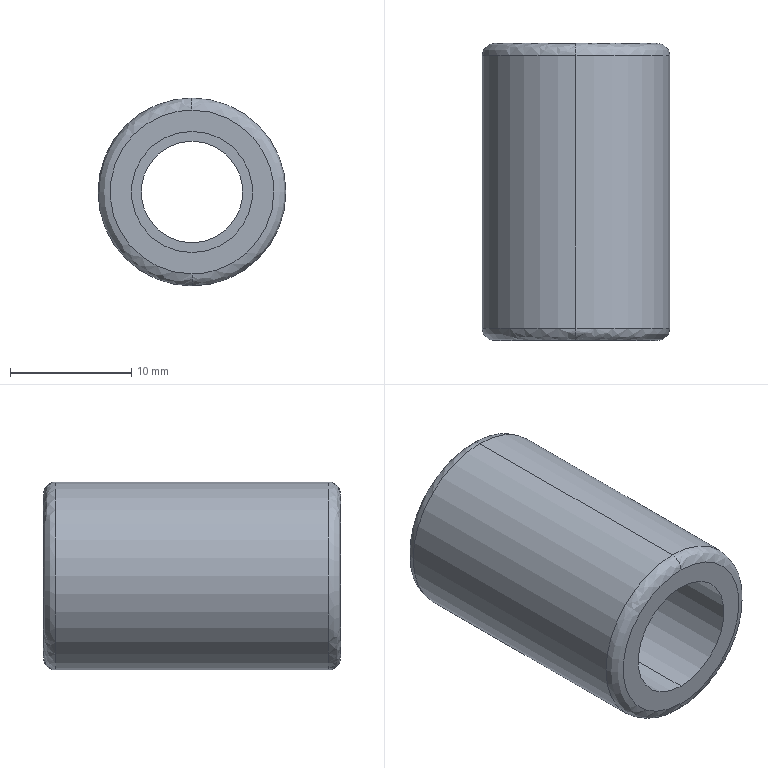Component | SolidWorks | SC-80x75(000)-1_11-1 | 1 solid | 27 faces | box 15.5 x 24.5 x 15.5 mm | volume 2654 mm3 | plane 15 | cylinder 6 | spline 4 | cone 2 | commonest cylinder face diameters 10 x2 15.5 x2 8.376 x2
STEP:
#1=COLOUR_RGB('',0.7922,0.8196,0.9333);
#2=FILL_AREA_STYLE_COLOUR('',#1);
#3=FILL_AREA_STYLE('',(#2));
#4=SURFACE_STYLE_FILL_AREA(#3);
#5=SURFACE_SIDE_STYLE('',(#4));
#6=SURFACE_STYLE_USAGE(.BOTH.,#5);
#7=PRESENTATION_STYLE_ASSIGNMENT((#6));
#8=CARTESIAN_POINT('',(-0.5951,7.131,9.518));
#9=VERTEX_POINT('',#8);
#10=CARTESIAN_POINT('',(-0.5951,7.131,8.986));
#11=VERTEX_POINT('',#10);
#12=CARTESIAN_POINT('',(-0.5951,7.131,9.518));
#13=CARTESIAN_POINT('',(-1.127,7.131,9.518));
#14=CARTESIAN_POINT('',(-1.127,7.131,8.986));
#15=CARTESIAN_POINT('',(-0.5951,7.131,8.986));
#16=(BOUNDED_CURVE()B_SPLINE_CURVE(3,(#12,#13,#14,#15),.UNSPECIFIED.,.F.,.F.)B_SPLINE_CURVE_WITH_KNOTS((4,4),(0.,1.),.UNSPECIFIED.)CURVE()GEOMETRIC_REPRESENTATION_ITEM()RATIONAL_B_SPLINE_CURVE((1.,0.3333,0.3333,1.))REPRESENTATION_ITEM(''));
#17=EDGE_CURVE('',#9,#11,#16,.T.);
#18=ORIENTED_EDGE('',*,*,#17,.T.);
#19=CARTESIAN_POINT('',(-0.5951,7.092,8.947));
#20=VERTEX_POINT('',#19);
#21=CARTESIAN_POINT('',(-0.5951,7.092,8.986));
#22=DIRECTION('',(-1.,-0.,-0.));
#23=DIRECTION('',(0.,0.,-1.));
#24=AXIS2_PLACEMENT_3D('',#21,#22,#23);
#25=CIRCLE('',#24,0.03937);
#26=EDGE_CURVE('',#11,#20,#25,.T.);
#27=ORIENTED_EDGE('',*,*,#26,.T.);
#28=CARTESIAN_POINT('',(-0.5951,7.092,9.557));
#29=VERTEX_POINT('',#28);
#30=CARTESIAN_POINT('',(-0.5951,7.092,9.252));
#31=DIRECTION('',(0.,-1.,0.));
#32=DIRECTION('',(-0.,0.,1.));
#33=AXIS2_PLACEMENT_3D('',#30,#31,#32);
#34=CIRCLE('',#33,0.3051);
#35=EDGE_CURVE('',#29,#20,#34,.T.);
#36=ORIENTED_EDGE('',*,*,#35,.F.);
#37=CARTESIAN_POINT('',(-0.5951,7.092,9.518));
#38=DIRECTION('',(1.,0.,0.));
#39=DIRECTION('',(0.,0.,1.));
#40=AXIS2_PLACEMENT_3D('',#37,#38,#39);
#41=CIRCLE('',#40,0.03937);
#42=EDGE_CURVE('',#9,#29,#41,.T.);
#43=ORIENTED_EDGE('',*,*,#42,.F.);
#44=EDGE_LOOP('',(#18,#27,#36,#43));
#45=FACE_OUTER_BOUND('',#44,.T.);
#46=CARTESIAN_POINT('',(-0.5951,7.131,8.986));
#47=CARTESIAN_POINT('',(-1.127,7.131,8.986));
#48=CARTESIAN_POINT('',(-1.127,7.131,9.518));
#49=CARTESIAN_POINT('',(-0.5951,7.131,9.518));
#50=CARTESIAN_POINT('',(-0.5951,7.131,8.963));
#51=CARTESIAN_POINT('',(-1.173,7.131,8.963));
#52=CARTESIAN_POINT('',(-1.173,7.131,9.541));
#53=CARTESIAN_POINT('',(-0.5951,7.131,9.541));
#54=CARTESIAN_POINT('',(-0.5951,7.115,8.947));
#55=CARTESIAN_POINT('',(-1.205,7.115,8.947));
#56=CARTESIAN_POINT('',(-1.205,7.115,9.557));
#57=CARTESIAN_POINT('',(-0.5951,7.115,9.557));
#58=CARTESIAN_POINT('',(-0.5951,7.092,8.947));
#59=CARTESIAN_POINT('',(-1.205,7.092,8.947));
#60=CARTESIAN_POINT('',(-1.205,7.092,9.557));
#61=CARTESIAN_POINT('',(-0.5951,7.092,9.557));
#62=(BOUNDED_SURFACE()B_SPLINE_SURFACE(3,3,((#46,#47,#48,#49),(#50,#51,#52,#53),(#54,#55,#56,#57),(#58,#59,#60,#61)),.UNSPECIFIED.,.F.,.F.,.T.)B_SPLINE_SURFACE_WITH_KNOTS((4,4),(4,4),(0.,1.),(0.,1.),.UNSPECIFIED.)GEOMETRIC_REPRESENTATION_ITEM()RATIONAL_B_SPLINE_SURFACE(((1.,0.3333,0.3333,1.),(0.8047,0.2682,0.2682,0.8047),(0.8047,0.2682,0.2682,0.8047),(1.,0.3333,0.3333,1.)))REPRESENTATION_ITEM('')SURFACE());
#63=ADVANCED_FACE('',(#45),#62,.T.);
#64=CARTESIAN_POINT('',(-0.5951,6.206,8.947));
#65=VERTEX_POINT('',#64);
#66=CARTESIAN_POINT('',(-0.5951,6.206,9.557));
#67=VERTEX_POINT('',#66);
#68=CARTESIAN_POINT('',(-0.5951,6.206,9.252));
#69=DIRECTION('',(-0.,1.,-0.));
#70=DIRECTION('',(-0.,0.,1.));
#71=AXIS2_PLACEMENT_3D('',#68,#69,#70);
#72=CIRCLE('',#71,0.3051);
#73=EDGE_CURVE('',#65,#67,#72,.T.);
#74=ORIENTED_EDGE('',*,*,#73,.F.);
#75=CARTESIAN_POINT('',(-0.5951,6.167,8.986));
#76=VERTEX_POINT('',#75);
#77=CARTESIAN_POINT('',(-0.5951,6.206,8.986));
#78=DIRECTION('',(-1.,-0.,-0.));
#79=DIRECTION('',(0.,0.,-1.));
#80=AXIS2_PLACEMENT_3D('',#77,#78,#79);
#81=CIRCLE('',#80,0.03937);
#82=EDGE_CURVE('',#65,#76,#81,.T.);
#83=ORIENTED_EDGE('',*,*,#82,.T.);
#84=CARTESIAN_POINT('',(-0.5951,6.167,9.518));
#85=VERTEX_POINT('',#84);
#86=CARTESIAN_POINT('',(-0.5951,6.167,8.986));
#87=CARTESIAN_POINT('',(-1.127,6.167,8.986));
#88=CARTESIAN_POINT('',(-1.127,6.167,9.518));
#89=CARTESIAN_POINT('',(-0.5951,6.167,9.518));
#90=(BOUNDED_CURVE()B_SPLINE_CURVE(3,(#86,#87,#88,#89),.UNSPECIFIED.,.F.,.F.)B_SPLINE_CURVE_WITH_KNOTS((4,4),(0.,1.),.UNSPECIFIED.)CURVE()GEOMETRIC_REPRESENTATION_ITEM()RATIONAL_B_SPLINE_CURVE((1.,0.3333,0.3333,1.))REPRESENTATION_ITEM(''));
#91=EDGE_CURVE('',#76,#85,#90,.T.);
#92=ORIENTED_EDGE('',*,*,#91,.T.);
#93=CARTESIAN_POINT('',(-0.5951,6.206,9.518));
#94=DIRECTION('',(1.,0.,0.));
#95=DIRECTION('',(0.,0.,1.));
#96=AXIS2_PLACEMENT_3D('',#93,#94,#95);
#97=CIRCLE('',#96,0.03937);
#98=EDGE_CURVE('',#67,#85,#97,.T.);
#99=ORIENTED_EDGE('',*,*,#98,.F.);
#100=EDGE_LOOP('',(#74,#83,#92,#99));
#101=FACE_OUTER_BOUND('',#100,.T.);
#102=CARTESIAN_POINT('',(-0.5951,6.206,8.947));
#103=CARTESIAN_POINT('',(-1.205,6.206,8.947));
#104=CARTESIAN_POINT('',(-1.205,6.206,9.557));
#105=CARTESIAN_POINT('',(-0.5951,6.206,9.557));
#106=CARTESIAN_POINT('',(-0.5951,6.183,8.947));
#107=CARTESIAN_POINT('',(-1.205,6.183,8.947));
#108=CARTESIAN_POINT('',(-1.205,6.183,9.557));
#109=CARTESIAN_POINT('',(-0.5951,6.183,9.557));
#110=CARTESIAN_POINT('',(-0.5951,6.167,8.963));
#111=CARTESIAN_POINT('',(-1.173,6.167,8.963));
#112=CARTESIAN_POINT('',(-1.173,6.167,9.541));
#113=CARTESIAN_POINT('',(-0.5951,6.167,9.541));
#114=CARTESIAN_POINT('',(-0.5951,6.167,8.986));
#115=CARTESIAN_POINT('',(-1.127,6.167,8.986));
#116=CARTESIAN_POINT('',(-1.127,6.167,9.518));
#117=CARTESIAN_POINT('',(-0.5951,6.167,9.518));
#118=(BOUNDED_SURFACE()B_SPLINE_SURFACE(3,3,((#102,#103,#104,#105),(#106,#107,#108,#109),(#110,#111,#112,#113),(#114,#115,#116,#117)),.UNSPECIFIED.,.F.,.F.,.T.)B_SPLINE_SURFACE_WITH_KNOTS((4,4),(4,4),(0.,1.),(0.,1.),.UNSPECIFIED.)GEOMETRIC_REPRESENTATION_ITEM()RATIONAL_B_SPLINE_SURFACE(((1.,0.3333,0.3333,1.),(0.8047,0.2682,0.2682,0.8047),(0.8047,0.2682,0.2682,0.8047),(1.,0.3333,0.3333,1.)))REPRESENTATION_ITEM('')SURFACE());
#119=ADVANCED_FACE('',(#101),#118,.T.);
#120=CARTESIAN_POINT('',(-0.5951,6.919,9.449));
#121=VERTEX_POINT('',#120);
#122=CARTESIAN_POINT('',(-0.5951,6.919,9.055));
#123=VERTEX_POINT('',#122);
#124=CARTESIAN_POINT('',(-0.5951,6.919,9.252));
#125=DIRECTION('',(-0.,1.,-0.));
#126=DIRECTION('',(0.,0.,-1.));
#127=AXIS2_PLACEMENT_3D('',#124,#125,#126);
#128=CIRCLE('',#127,0.1969);
#129=EDGE_CURVE('',#121,#123,#128,.T.);
#130=ORIENTED_EDGE('',*,*,#129,.T.);
#131=CARTESIAN_POINT('',(-0.5951,6.167,9.055));
#132=VERTEX_POINT('',#131);
#133=CARTESIAN_POINT('',(-0.5951,6.919,9.055));
#134=DIRECTION('',(0.,-1.,0.));
#135=VECTOR('',#134,39.37);
#136=LINE('',#133,#135);
#137=EDGE_CURVE('',#123,#132,#136,.T.);
#138=ORIENTED_EDGE('',*,*,#137,.T.);
#139=CARTESIAN_POINT('',(-0.5951,6.167,9.449));
#140=VERTEX_POINT('',#139);
#141=CARTESIAN_POINT('',(-0.5951,6.167,9.252));
#142=DIRECTION('',(-0.,1.,-0.));
#143=DIRECTION('',(1.,0.,0.));
#144=AXIS2_PLACEMENT_3D('',#141,#142,#143);
#145=CIRCLE('',#144,0.1969);
#146=EDGE_CURVE('',#140,#132,#145,.T.);
#147=ORIENTED_EDGE('',*,*,#146,.F.);
#148=CARTESIAN_POINT('',(-0.5951,6.919,9.449));
#149=DIRECTION('',(0.,-1.,0.));
#150=VECTOR('',#149,39.37);
#151=LINE('',#148,#150);
#152=EDGE_CURVE('',#121,#140,#151,.T.);
#153=ORIENTED_EDGE('',*,*,#152,.F.);
#154=EDGE_LOOP('',(#130,#138,#147,#153));
#155=FACE_OUTER_BOUND('',#154,.T.);
#156=CARTESIAN_POINT('',(-0.5951,6.919,9.252));
#157=DIRECTION('',(0.,-1.,0.));
#158=DIRECTION('',(-0.,0.,1.));
#159=AXIS2_PLACEMENT_3D('',#156,#157,#158);
#160=CYLINDRICAL_SURFACE('',#159,0.1969);
#161=ADVANCED_FACE('',(#155),#160,.F.);
#162=ORIENTED_EDGE('',*,*,#35,.T.);
#163=CARTESIAN_POINT('',(-0.5951,6.649,8.947));
#164=DIRECTION('',(0.,-1.,0.));
#165=VECTOR('',#164,39.37);
#166=LINE('',#163,#165);
#167=EDGE_CURVE('',#20,#65,#166,.T.);
#168=ORIENTED_EDGE('',*,*,#167,.T.);
#169=ORIENTED_EDGE('',*,*,#73,.T.);
#170=CARTESIAN_POINT('',(-0.5951,6.649,9.557));
#171=DIRECTION('',(0.,-1.,0.));
#172=VECTOR('',#171,39.37);
#173=LINE('',#170,#172);
#174=EDGE_CURVE('',#29,#67,#173,.T.);
#175=ORIENTED_EDGE('',*,*,#174,.F.);
#176=EDGE_LOOP('',(#162,#168,#169,#175));
#177=FACE_OUTER_BOUND('',#176,.T.);
#178=CARTESIAN_POINT('',(-0.5951,6.649,9.252));
#179=DIRECTION('',(0.,-1.,0.));
#180=DIRECTION('',(-0.,0.,1.));
#181=AXIS2_PLACEMENT_3D('',#178,#179,#180);
#182=CYLINDRICAL_SURFACE('',#181,0.3051);
#183=ADVANCED_FACE('',(#177),#182,.T.);
#184=CARTESIAN_POINT('',(-0.5951,6.922,9.087));
#185=VERTEX_POINT('',#184);
#186=CARTESIAN_POINT('',(-0.5951,6.922,9.417));
#187=VERTEX_POINT('',#186);
#188=CARTESIAN_POINT('',(-0.5951,6.922,9.252));
#189=DIRECTION('',(0.,-1.,0.));
#190=DIRECTION('',(-0.,0.,1.));
#191=AXIS2_PLACEMENT_3D('',#188,#189,#190);
#192=CIRCLE('',#191,0.1649);
#193=EDGE_CURVE('',#185,#187,#192,.T.);
#194=ORIENTED_EDGE('',*,*,#193,.F.);
#195=CARTESIAN_POINT('',(-0.5951,6.919,9.087));
#196=VERTEX_POINT('',#195);
#197=CARTESIAN_POINT('',(-0.5951,6.561,9.087));
#198=DIRECTION('',(0.,-1.,0.));
#199=VECTOR('',#198,39.37);
#200=LINE('',#197,#199);
#201=EDGE_CURVE('',#185,#196,#200,.T.);
#202=ORIENTED_EDGE('',*,*,#201,.T.);
#203=CARTESIAN_POINT('',(-0.5951,6.919,9.417));
#204=VERTEX_POINT('',#203);
#205=CARTESIAN_POINT('',(-0.5951,6.919,9.252));
#206=DIRECTION('',(0.,-1.,0.));
#207=DIRECTION('',(0.,0.,-1.));
#208=AXIS2_PLACEMENT_3D('',#205,#206,#207);
#209=CIRCLE('',#208,0.1649);
#210=EDGE_CURVE('',#196,#204,#209,.T.);
#211=ORIENTED_EDGE('',*,*,#210,.T.);
#212=CARTESIAN_POINT('',(-0.5951,6.561,9.417));
#213=DIRECTION('',(0.,-1.,0.));
#214=VECTOR('',#213,39.37);
#215=LINE('',#212,#214);
#216=EDGE_CURVE('',#187,#204,#215,.T.);
#217=ORIENTED_EDGE('',*,*,#216,.F.);
#218=EDGE_LOOP('',(#194,#202,#211,#217));
#219=FACE_OUTER_BOUND('',#218,.T.);
#220=CARTESIAN_POINT('',(-0.5951,6.561,9.252));
#221=DIRECTION('',(0.,-1.,0.));
#222=DIRECTION('',(-0.,0.,1.));
#223=AXIS2_PLACEMENT_3D('',#220,#221,#222);
#224=CYLINDRICAL_SURFACE('',#223,0.1649);
#225=ADVANCED_FACE('',(#219),#224,.F.);
#226=ORIENTED_EDGE('',*,*,#193,.T.);
#227=CARTESIAN_POINT('',(-0.5951,6.954,9.449));
#228=VERTEX_POINT('',#227);
#229=CARTESIAN_POINT('',(-0.5951,6.954,9.449));
#230=DIRECTION('',(-0.,0.7071,0.7071));
#231=VECTOR('',#230,39.37);
#232=LINE('',#229,#231);
#233=EDGE_CURVE('',#187,#228,#232,.T.);
#234=ORIENTED_EDGE('',*,*,#233,.T.);
#235=CARTESIAN_POINT('',(-0.4246,6.954,9.35));
#236=VERTEX_POINT('',#235);
#237=CARTESIAN_POINT('',(-0.5951,6.954,9.252));
#238=DIRECTION('',(-0.,1.,-0.));
#239=DIRECTION('',(0.,0.,-1.));
#240=AXIS2_PLACEMENT_3D('',#237,#238,#239);
#241=CIRCLE('',#240,0.1969);
#242=EDGE_CURVE('',#228,#236,#241,.T.);
#243=ORIENTED_EDGE('',*,*,#242,.T.);
#244=CARTESIAN_POINT('',(-0.4246,6.954,9.154));
#245=VERTEX_POINT('',#244);
#246=CARTESIAN_POINT('',(-0.5951,6.954,9.252));
#247=DIRECTION('',(-0.,1.,-0.));
#248=DIRECTION('',(0.,0.,-1.));
#249=AXIS2_PLACEMENT_3D('',#246,#247,#248);
#250=CIRCLE('',#249,0.1969);
#251=EDGE_CURVE('',#236,#245,#250,.T.);
#252=ORIENTED_EDGE('',*,*,#251,.T.);
#253=CARTESIAN_POINT('',(-0.5951,6.954,9.055));
#254=VERTEX_POINT('',#253);
#255=CARTESIAN_POINT('',(-0.5951,6.954,9.252));
#256=DIRECTION('',(-0.,1.,-0.));
#257=DIRECTION('',(0.,0.,-1.));
#258=AXIS2_PLACEMENT_3D('',#255,#256,#257);
#259=CIRCLE('',#258,0.1969);
#260=EDGE_CURVE('',#245,#254,#259,.T.);
#261=ORIENTED_EDGE('',*,*,#260,.T.);
#262=CARTESIAN_POINT('',(-0.5951,6.954,9.055));
#263=DIRECTION('',(0.,0.7071,-0.7071));
#264=VECTOR('',#263,39.37);
#265=LINE('',#262,#264);
#266=EDGE_CURVE('',#185,#254,#265,.T.);
#267=ORIENTED_EDGE('',*,*,#266,.F.);
#268=EDGE_LOOP('',(#226,#234,#243,#252,#261,#267));
#269=FACE_OUTER_BOUND('',#268,.T.);
#270=CARTESIAN_POINT('',(-0.5951,6.954,9.252));
#271=DIRECTION('',(-0.,1.,-0.));
#272=DIRECTION('',(0.,0.,-1.));
#273=AXIS2_PLACEMENT_3D('',#270,#271,#272);
#274=CONICAL_SURFACE('',#273,0.1969,0.7854);
#275=ADVANCED_FACE('',(#269),#274,.F.);
#276=ORIENTED_EDGE('',*,*,#167,.F.);
#277=CARTESIAN_POINT('',(-0.5951,7.092,9.252));
#278=DIRECTION('',(0.,-1.,0.));
#279=DIRECTION('',(-0.,0.,1.));
#280=AXIS2_PLACEMENT_3D('',#277,#278,#279);
#281=CIRCLE('',#280,0.3051);
#282=EDGE_CURVE('',#20,#29,#281,.T.);
#283=ORIENTED_EDGE('',*,*,#282,.T.);
#284=ORIENTED_EDGE('',*,*,#174,.T.);
#285=CARTESIAN_POINT('',(-0.5951,6.206,9.252));
#286=DIRECTION('',(-0.,1.,-0.));
#287=DIRECTION('',(-0.,0.,1.));
#288=AXIS2_PLACEMENT_3D('',#285,#286,#287);
#289=CIRCLE('',#288,0.3051);
#290=EDGE_CURVE('',#67,#65,#289,.T.);
#291=ORIENTED_EDGE('',*,*,#290,.T.);
#292=EDGE_LOOP('',(#276,#283,#284,#291));
#293=FACE_OUTER_BOUND('',#292,.T.);
#294=CARTESIAN_POINT('',(-0.5951,6.649,9.252));
#295=DIRECTION('',(0.,-1.,0.));
#296=DIRECTION('',(-0.,0.,1.));
#297=AXIS2_PLACEMENT_3D('',#294,#295,#296);
#298=CYLINDRICAL_SURFACE('',#297,0.3051);
#299=ADVANCED_FACE('',(#293),#298,.T.);
#300=ORIENTED_EDGE('',*,*,#26,.F.);
#301=CARTESIAN_POINT('',(-0.3294,7.131,9.252));
#302=VERTEX_POINT('',#301);
#303=CARTESIAN_POINT('',(-0.5951,7.131,8.986));
#304=CARTESIAN_POINT('',(-0.4394,7.131,8.986));
#305=CARTESIAN_POINT('',(-0.3294,7.131,9.096));
#306=CARTESIAN_POINT('',(-0.3294,7.131,9.252));
#307=(BOUNDED_CURVE()B_SPLINE_CURVE(3,(#303,#304,#305,#306),.UNSPECIFIED.,.F.,.T.)B_SPLINE_CURVE_WITH_KNOTS((4,4),(0.,1.),.UNSPECIFIED.)CURVE()GEOMETRIC_REPRESENTATION_ITEM()RATIONAL_B_SPLINE_CURVE((1.,0.8047,0.8047,1.))REPRESENTATION_ITEM(''));
#308=EDGE_CURVE('',#11,#302,#307,.T.);
#309=ORIENTED_EDGE('',*,*,#308,.T.);
#310=CARTESIAN_POINT('',(-0.3294,7.131,9.252));
#311=CARTESIAN_POINT('',(-0.3294,7.131,9.408));
#312=CARTESIAN_POINT('',(-0.4394,7.131,9.518));
#313=CARTESIAN_POINT('',(-0.5951,7.131,9.518));
#314=(BOUNDED_CURVE()B_SPLINE_CURVE(3,(#310,#311,#312,#313),.UNSPECIFIED.,.F.,.T.)B_SPLINE_CURVE_WITH_KNOTS((4,4),(0.,1.),.UNSPECIFIED.)CURVE()GEOMETRIC_REPRESENTATION_ITEM()RATIONAL_B_SPLINE_CURVE((1.,0.8047,0.8047,1.))REPRESENTATION_ITEM(''));
#315=EDGE_CURVE('',#302,#9,#314,.T.);
#316=ORIENTED_EDGE('',*,*,#315,.T.);
#317=ORIENTED_EDGE('',*,*,#42,.T.);
#318=ORIENTED_EDGE('',*,*,#282,.F.);
#319=EDGE_LOOP('',(#300,#309,#316,#317,#318));
#320=FACE_OUTER_BOUND('',#319,.T.);
#321=CARTESIAN_POINT('',(-0.5951,7.131,9.518));
#322=CARTESIAN_POINT('',(-0.06362,7.131,9.518));
#323=CARTESIAN_POINT('',(-0.06362,7.131,8.986));
#324=CARTESIAN_POINT('',(-0.5951,7.131,8.986));
#325=CARTESIAN_POINT('',(-0.5951,7.131,9.541));
#326=CARTESIAN_POINT('',(-0.01749,7.131,9.541));
#327=CARTESIAN_POINT('',(-0.01749,7.131,8.963));
#328=CARTESIAN_POINT('',(-0.5951,7.131,8.963));
#329=CARTESIAN_POINT('',(-0.5951,7.115,9.557));
#330=CARTESIAN_POINT('',(0.01512,7.115,9.557));
#331=CARTESIAN_POINT('',(0.01512,7.115,8.947));
#332=CARTESIAN_POINT('',(-0.5951,7.115,8.947));
#333=CARTESIAN_POINT('',(-0.5951,7.092,9.557));
#334=CARTESIAN_POINT('',(0.01512,7.092,9.557));
#335=CARTESIAN_POINT('',(0.01512,7.092,8.947));
#336=CARTESIAN_POINT('',(-0.5951,7.092,8.947));
#337=(BOUNDED_SURFACE()B_SPLINE_SURFACE(3,3,((#321,#322,#323,#324),(#325,#326,#327,#328),(#329,#330,#331,#332),(#333,#334,#335,#336)),.UNSPECIFIED.,.F.,.F.,.T.)B_SPLINE_SURFACE_WITH_KNOTS((4,4),(4,4),(0.,1.),(0.,1.),.UNSPECIFIED.)GEOMETRIC_REPRESENTATION_ITEM()RATIONAL_B_SPLINE_SURFACE(((1.,0.3333,0.3333,1.),(0.8047,0.2682,0.2682,0.8047),(0.8047,0.2682,0.2682,0.8047),(1.,0.3333,0.3333,1.)))REPRESENTATION_ITEM('')SURFACE());
#338=ADVANCED_FACE('',(#320),#337,.T.);
#339=ORIENTED_EDGE('',*,*,#82,.F.);
#340=ORIENTED_EDGE('',*,*,#290,.F.);
#341=ORIENTED_EDGE('',*,*,#98,.T.);
#342=CARTESIAN_POINT('',(-0.3294,6.167,9.252));
#343=VERTEX_POINT('',#342);
#344=CARTESIAN_POINT('',(-0.5951,6.167,9.518));
#345=CARTESIAN_POINT('',(-0.4394,6.167,9.518));
#346=CARTESIAN_POINT('',(-0.3294,6.167,9.408));
#347=CARTESIAN_POINT('',(-0.3294,6.167,9.252));
#348=(BOUNDED_CURVE()B_SPLINE_CURVE(3,(#344,#345,#346,#347),.UNSPECIFIED.,.F.,.F.)B_SPLINE_CURVE_WITH_KNOTS((4,4),(0.,1.),.UNSPECIFIED.)CURVE()GEOMETRIC_REPRESENTATION_ITEM()RATIONAL_B_SPLINE_CURVE((1.,0.8047,0.8047,1.))REPRESENTATION_ITEM(''));
#349=EDGE_CURVE('',#85,#343,#348,.T.);
#350=ORIENTED_EDGE('',*,*,#349,.T.);
#351=CARTESIAN_POINT('',(-0.3294,6.167,9.252));
#352=CARTESIAN_POINT('',(-0.3294,6.167,9.096));
#353=CARTESIAN_POINT('',(-0.4394,6.167,8.986));
#354=CARTESIAN_POINT('',(-0.5951,6.167,8.986));
#355=(BOUNDED_CURVE()B_SPLINE_CURVE(3,(#351,#352,#353,#354),.UNSPECIFIED.,.F.,.F.)B_SPLINE_CURVE_WITH_KNOTS((4,4),(0.,1.),.UNSPECIFIED.)CURVE()GEOMETRIC_REPRESENTATION_ITEM()RATIONAL_B_SPLINE_CURVE((1.,0.8047,0.8047,1.))REPRESENTATION_ITEM(''));
#356=EDGE_CURVE('',#343,#76,#355,.T.);
#357=ORIENTED_EDGE('',*,*,#356,.T.);
#358=EDGE_LOOP('',(#339,#340,#341,#350,#357));
#359=FACE_OUTER_BOUND('',#358,.T.);
#360=CARTESIAN_POINT('',(-0.5951,6.206,9.557));
#361=CARTESIAN_POINT('',(0.01512,6.206,9.557));
#362=CARTESIAN_POINT('',(0.01512,6.206,8.947));
#363=CARTESIAN_POINT('',(-0.5951,6.206,8.947));
#364=CARTESIAN_POINT('',(-0.5951,6.183,9.557));
#365=CARTESIAN_POINT('',(0.01512,6.183,9.557));
#366=CARTESIAN_POINT('',(0.01512,6.183,8.947));
#367=CARTESIAN_POINT('',(-0.5951,6.183,8.947));
#368=CARTESIAN_POINT('',(-0.5951,6.167,9.541));
#369=CARTESIAN_POINT('',(-0.01749,6.167,9.541));
#370=CARTESIAN_POINT('',(-0.01749,6.167,8.963));
#371=CARTESIAN_POINT('',(-0.5951,6.167,8.963));
#372=CARTESIAN_POINT('',(-0.5951,6.167,9.518));
#373=CARTESIAN_POINT('',(-0.06362,6.167,9.518));
#374=CARTESIAN_POINT('',(-0.06362,6.167,8.986));
#375=CARTESIAN_POINT('',(-0.5951,6.167,8.986));
#376=(BOUNDED_SURFACE()B_SPLINE_SURFACE(3,3,((#360,#361,#362,#363),(#364,#365,#366,#367),(#368,#369,#370,#371),(#372,#373,#374,#375)),.UNSPECIFIED.,.F.,.F.,.T.)B_SPLINE_SURFACE_WITH_KNOTS((4,4),(4,4),(0.,1.),(0.,1.),.UNSPECIFIED.)GEOMETRIC_REPRESENTATION_ITEM()RATIONAL_B_SPLINE_SURFACE(((1.,0.3333,0.3333,1.),(0.8047,0.2682,0.2682,0.8047),(0.8047,0.2682,0.2682,0.8047),(1.,0.3333,0.3333,1.)))REPRESENTATION_ITEM('')SURFACE());
#377=ADVANCED_FACE('',(#359),#376,.T.);
#378=ORIENTED_EDGE('',*,*,#17,.F.);
#379=ORIENTED_EDGE('',*,*,#315,.F.);
#380=ORIENTED_EDGE('',*,*,#308,.F.);
#381=EDGE_LOOP('',(#378,#379,#380));
#382=FACE_OUTER_BOUND('',#381,.T.);
#383=CARTESIAN_POINT('',(-0.7088,7.131,9.055));
#384=VERTEX_POINT('',#383);
#385=CARTESIAN_POINT('',(-0.4815,7.131,9.055));
#386=VERTEX_POINT('',#385);
#387=CARTESIAN_POINT('',(-0.4622,7.131,9.055));
#388=DIRECTION('',(1.,0.,0.));
#389=VECTOR('',#388,39.37);
#390=LINE('',#387,#389);
#391=EDGE_CURVE('',#384,#386,#390,.T.);
#392=ORIENTED_EDGE('',*,*,#391,.T.);
#393=CARTESIAN_POINT('',(-0.3678,7.131,9.252));
#394=VERTEX_POINT('',#393);
#395=CARTESIAN_POINT('',(-0.4815,7.131,9.055));
#396=DIRECTION('',(0.5,0.,0.866));
#397=VECTOR('',#396,39.37);
#398=LINE('',#395,#397);
#399=EDGE_CURVE('',#386,#394,#398,.T.);
#400=ORIENTED_EDGE('',*,*,#399,.T.);
#401=CARTESIAN_POINT('',(-0.4815,7.131,9.449));
#402=VERTEX_POINT('',#401);
#403=CARTESIAN_POINT('',(-0.3678,7.131,9.252));
#404=DIRECTION('',(-0.5,-0.,0.866));
#405=VECTOR('',#404,39.37);
#406=LINE('',#403,#405);
#407=EDGE_CURVE('',#394,#402,#406,.T.);
#408=ORIENTED_EDGE('',*,*,#407,.T.);
#409=CARTESIAN_POINT('',(-0.7088,7.131,9.449));
#410=VERTEX_POINT('',#409);
#411=CARTESIAN_POINT('',(-0.4622,7.131,9.449));
#412=DIRECTION('',(-1.,-0.,-0.));
#413=VECTOR('',#412,39.37);
#414=LINE('',#411,#413);
#415=EDGE_CURVE('',#402,#410,#414,.T.);
#416=ORIENTED_EDGE('',*,*,#415,.T.);
#417=CARTESIAN_POINT('',(-0.8224,7.131,9.252));
#418=VERTEX_POINT('',#417);
#419=CARTESIAN_POINT('',(-0.7088,7.131,9.449));
#420=DIRECTION('',(-0.5,-0.,-0.866));
#421=VECTOR('',#420,39.37);
#422=LINE('',#419,#421);
#423=EDGE_CURVE('',#410,#418,#422,.T.);
#424=ORIENTED_EDGE('',*,*,#423,.T.);
#425=CARTESIAN_POINT('',(-0.8224,7.131,9.252));
#426=DIRECTION('',(0.5,0.,-0.866));
#427=VECTOR('',#426,39.37);
#428=LINE('',#425,#427);
#429=EDGE_CURVE('',#418,#384,#428,.T.);
#430=ORIENTED_EDGE('',*,*,#429,.T.);
#431=EDGE_LOOP('',(#392,#400,#408,#416,#424,#430));
#432=FACE_BOUND('',#431,.T.);
#433=CARTESIAN_POINT('',(-0.4622,7.131,9.252));
#434=DIRECTION('',(-0.,1.,-0.));
#435=DIRECTION('',(0.,0.,-1.));
#436=AXIS2_PLACEMENT_3D('',#433,#434,#435);
#437=PLANE('',#436);
#438=ADVANCED_FACE('',(#382,#432),#437,.T.);
#439=ORIENTED_EDGE('',*,*,#349,.F.);
#440=ORIENTED_EDGE('',*,*,#91,.F.);
#441=ORIENTED_EDGE('',*,*,#356,.F.);
#442=EDGE_LOOP('',(#439,#440,#441));
#443=FACE_OUTER_BOUND('',#442,.T.);
#444=ORIENTED_EDGE('',*,*,#146,.T.);
#445=CARTESIAN_POINT('',(-0.5951,6.167,9.252));
#446=DIRECTION('',(-0.,1.,-0.));
#447=DIRECTION('',(1.,0.,0.));
#448=AXIS2_PLACEMENT_3D('',#445,#446,#447);
#449=CIRCLE('',#448,0.1969);
#450=EDGE_CURVE('',#132,#140,#449,.T.);
#451=ORIENTED_EDGE('',*,*,#450,.T.);
#452=EDGE_LOOP('',(#444,#451));
#453=FACE_BOUND('',#452,.T.);
#454=CARTESIAN_POINT('',(-0.4622,6.167,9.252));
#455=DIRECTION('',(0.,-1.,0.));
#456=DIRECTION('',(1.,0.,0.));
#457=AXIS2_PLACEMENT_3D('',#454,#455,#456);
#458=PLANE('',#457);
#459=ADVANCED_FACE('',(#443,#453),#458,.T.);
#460=CARTESIAN_POINT('',(-0.3678,6.954,9.252));
#461=VERTEX_POINT('',#460);
#462=CARTESIAN_POINT('',(-0.3678,7.131,9.252));
#463=DIRECTION('',(0.,-1.,0.));
#464=VECTOR('',#463,39.37);
#465=LINE('',#462,#464);
#466=EDGE_CURVE('',#394,#461,#465,.T.);
#467=ORIENTED_EDGE('',*,*,#466,.F.);
#468=ORIENTED_EDGE('',*,*,#399,.F.);
#469=CARTESIAN_POINT('',(-0.4815,6.954,9.055));
#470=VERTEX_POINT('',#469);
#471=CARTESIAN_POINT('',(-0.4815,7.131,9.055));
#472=DIRECTION('',(-0.,1.,-0.));
#473=VECTOR('',#472,39.37);
#474=LINE('',#471,#473);
#475=EDGE_CURVE('',#470,#386,#474,.T.);
#476=ORIENTED_EDGE('',*,*,#475,.F.);
#477=CARTESIAN_POINT('',(-0.3678,6.954,9.252));
#478=DIRECTION('',(-0.5,-0.,-0.866));
#479=VECTOR('',#478,39.37);
#480=LINE('',#477,#479);
#481=EDGE_CURVE('',#245,#470,#480,.T.);
#482=ORIENTED_EDGE('',*,*,#481,.F.);
#483=CARTESIAN_POINT('',(-0.3678,6.954,9.252));
#484=DIRECTION('',(-0.5,-0.,-0.866));
#485=VECTOR('',#484,39.37);
#486=LINE('',#483,#485);
#487=EDGE_CURVE('',#461,#245,#486,.T.);
#488=ORIENTED_EDGE('',*,*,#487,.F.);
#489=EDGE_LOOP('',(#467,#468,#476,#482,#488));
#490=FACE_OUTER_BOUND('',#489,.T.);
#491=CARTESIAN_POINT('',(-0.3678,7.131,9.252));
#492=DIRECTION('',(0.866,0.,-0.5));
#493=DIRECTION('',(-0.5,-0.,-0.866));
#494=AXIS2_PLACEMENT_3D('',#491,#492,#493);
#495=PLANE('',#494);
#496=ADVANCED_FACE('',(#490),#495,.F.);
#497=ORIENTED_EDGE('',*,*,#475,.T.);
#498=ORIENTED_EDGE('',*,*,#391,.F.);
#499=CARTESIAN_POINT('',(-0.7088,6.954,9.055));
#500=VERTEX_POINT('',#499);
#501=CARTESIAN_POINT('',(-0.7088,7.131,9.055));
#502=DIRECTION('',(-0.,1.,-0.));
#503=VECTOR('',#502,39.37);
#504=LINE('',#501,#503);
#505=EDGE_CURVE('',#500,#384,#504,.T.);
#506=ORIENTED_EDGE('',*,*,#505,.F.);
#507=CARTESIAN_POINT('',(-0.4815,6.954,9.055));
#508=DIRECTION('',(-1.,-0.,-0.));
#509=VECTOR('',#508,39.37);
#510=LINE('',#507,#509);
#511=EDGE_CURVE('',#254,#500,#510,.T.);
#512=ORIENTED_EDGE('',*,*,#511,.F.);
#513=CARTESIAN_POINT('',(-0.4815,6.954,9.055));
#514=DIRECTION('',(-1.,-0.,-0.));
#515=VECTOR('',#514,39.37);
#516=LINE('',#513,#515);
#517=EDGE_CURVE('',#470,#254,#516,.T.);
#518=ORIENTED_EDGE('',*,*,#517,.F.);
#519=EDGE_LOOP('',(#497,#498,#506,#512,#518));
#520=FACE_OUTER_BOUND('',#519,.T.);
#521=CARTESIAN_POINT('',(-0.4815,7.131,9.055));
#522=DIRECTION('',(0.,0.,-1.));
#523=DIRECTION('',(0.,-1.,0.));
#524=AXIS2_PLACEMENT_3D('',#521,#522,#523);
#525=PLANE('',#524);
#526=ADVANCED_FACE('',(#520),#525,.F.);
#527=ORIENTED_EDGE('',*,*,#505,.T.);
#528=ORIENTED_EDGE('',*,*,#429,.F.);
#529=CARTESIAN_POINT('',(-0.8224,6.954,9.252));
#530=VERTEX_POINT('',#529);
#531=CARTESIAN_POINT('',(-0.8224,7.131,9.252));
#532=DIRECTION('',(-0.,1.,-0.));
#533=VECTOR('',#532,39.37);
#534=LINE('',#531,#533);
#535=EDGE_CURVE('',#530,#418,#534,.T.);
#536=ORIENTED_EDGE('',*,*,#535,.F.);
#537=CARTESIAN_POINT('',(-0.7656,6.954,9.154));
#538=VERTEX_POINT('',#537);
#539=CARTESIAN_POINT('',(-0.7088,6.954,9.055));
#540=DIRECTION('',(-0.5,-0.,0.866));
#541=VECTOR('',#540,39.37);
#542=LINE('',#539,#541);
#543=EDGE_CURVE('',#538,#530,#542,.T.);
#544=ORIENTED_EDGE('',*,*,#543,.F.);
#545=CARTESIAN_POINT('',(-0.7088,6.954,9.055));
#546=DIRECTION('',(-0.5,-0.,0.866));
#547=VECTOR('',#546,39.37);
#548=LINE('',#545,#547);
#549=EDGE_CURVE('',#500,#538,#548,.T.);
#550=ORIENTED_EDGE('',*,*,#549,.F.);
#551=EDGE_LOOP('',(#527,#528,#536,#544,#550));
#552=FACE_OUTER_BOUND('',#551,.T.);
#553=CARTESIAN_POINT('',(-0.7088,7.131,9.055));
#554=DIRECTION('',(-0.866,-0.,-0.5));
#555=DIRECTION('',(-0.5,-0.,0.866));
#556=AXIS2_PLACEMENT_3D('',#553,#554,#555);
#557=PLANE('',#556);
#558=ADVANCED_FACE('',(#552),#557,.F.);
#559=ORIENTED_EDGE('',*,*,#535,.T.);
#560=ORIENTED_EDGE('',*,*,#423,.F.);
#561=CARTESIAN_POINT('',(-0.7088,6.954,9.449));
#562=VERTEX_POINT('',#561);
#563=CARTESIAN_POINT('',(-0.7088,7.131,9.449));
#564=DIRECTION('',(-0.,1.,-0.));
#565=VECTOR('',#564,39.37);
#566=LINE('',#563,#565);
#567=EDGE_CURVE('',#562,#410,#566,.T.);
#568=ORIENTED_EDGE('',*,*,#567,.F.);
#569=CARTESIAN_POINT('',(-0.7656,6.954,9.35));
#570=VERTEX_POINT('',#569);
#571=CARTESIAN_POINT('',(-0.8224,6.954,9.252));
#572=DIRECTION('',(0.5,0.,0.866));
#573=VECTOR('',#572,39.37);
#574=LINE('',#571,#573);
#575=EDGE_CURVE('',#570,#562,#574,.T.);
#576=ORIENTED_EDGE('',*,*,#575,.F.);
#577=CARTESIAN_POINT('',(-0.8224,6.954,9.252));
#578=DIRECTION('',(0.5,0.,0.866));
#579=VECTOR('',#578,39.37);
#580=LINE('',#577,#579);
#581=EDGE_CURVE('',#530,#570,#580,.T.);
#582=ORIENTED_EDGE('',*,*,#581,.F.);
#583=EDGE_LOOP('',(#559,#560,#568,#576,#582));
#584=FACE_OUTER_BOUND('',#583,.T.);
#585=CARTESIAN_POINT('',(-0.8224,7.131,9.252));
#586=DIRECTION('',(-0.866,-0.,0.5));
#587=DIRECTION('',(0.5,0.,0.866));
#588=AXIS2_PLACEMENT_3D('',#585,#586,#587);
#589=PLANE('',#588);
#590=ADVANCED_FACE('',(#584),#589,.F.);
#591=ORIENTED_EDGE('',*,*,#567,.T.);
#592=ORIENTED_EDGE('',*,*,#415,.F.);
#593=CARTESIAN_POINT('',(-0.4815,6.954,9.449));
#594=VERTEX_POINT('',#593);
#595=CARTESIAN_POINT('',(-0.4815,7.131,9.449));
#596=DIRECTION('',(-0.,1.,-0.));
#597=VECTOR('',#596,39.37);
#598=LINE('',#595,#597);
#599=EDGE_CURVE('',#594,#402,#598,.T.);
#600=ORIENTED_EDGE('',*,*,#599,.F.);
#601=CARTESIAN_POINT('',(-0.7088,6.954,9.449));
#602=DIRECTION('',(1.,0.,0.));
#603=VECTOR('',#602,39.37);
#604=LINE('',#601,#603);
#605=EDGE_CURVE('',#228,#594,#604,.T.);
#606=ORIENTED_EDGE('',*,*,#605,.F.);
#607=CARTESIAN_POINT('',(-0.7088,6.954,9.449));
#608=DIRECTION('',(1.,0.,0.));
#609=VECTOR('',#608,39.37);
#610=LINE('',#607,#609);
#611=EDGE_CURVE('',#562,#228,#610,.T.);
#612=ORIENTED_EDGE('',*,*,#611,.F.);
#613=EDGE_LOOP('',(#591,#592,#600,#606,#612));
#614=FACE_OUTER_BOUND('',#613,.T.);
#615=CARTESIAN_POINT('',(-0.7088,7.131,9.449));
#616=DIRECTION('',(-0.,-0.,1.));
#617=DIRECTION('',(-0.,1.,-0.));
#618=AXIS2_PLACEMENT_3D('',#615,#616,#617);
#619=PLANE('',#618);
#620=ADVANCED_FACE('',(#614),#619,.F.);
#621=ORIENTED_EDGE('',*,*,#599,.T.);
#622=ORIENTED_EDGE('',*,*,#407,.F.);
#623=ORIENTED_EDGE('',*,*,#466,.T.);
#624=CARTESIAN_POINT('',(-0.4815,6.954,9.449));
#625=DIRECTION('',(0.5,0.,-0.866));
#626=VECTOR('',#625,39.37);
#627=LINE('',#624,#626);
#628=EDGE_CURVE('',#236,#461,#627,.T.);
#629=ORIENTED_EDGE('',*,*,#628,.F.);
#630=CARTESIAN_POINT('',(-0.4815,6.954,9.449));
#631=DIRECTION('',(0.5,0.,-0.866));
#632=VECTOR('',#631,39.37);
#633=LINE('',#630,#632);
#634=EDGE_CURVE('',#594,#236,#633,.T.);
#635=ORIENTED_EDGE('',*,*,#634,.F.);
#636=EDGE_LOOP('',(#621,#622,#623,#629,#635));
#637=FACE_OUTER_BOUND('',#636,.T.);
#638=CARTESIAN_POINT('',(-0.4815,7.131,9.449));
#639=DIRECTION('',(0.866,0.,0.5));
#640=DIRECTION('',(0.5,0.,-0.866));
#641=AXIS2_PLACEMENT_3D('',#638,#639,#640);
#642=PLANE('',#641);
#643=ADVANCED_FACE('',(#637),#642,.F.);
#644=ORIENTED_EDGE('',*,*,#251,.F.);
#645=ORIENTED_EDGE('',*,*,#628,.T.);
#646=ORIENTED_EDGE('',*,*,#487,.T.);
#647=EDGE_LOOP('',(#644,#645,#646));
#648=FACE_OUTER_BOUND('',#647,.T.);
#649=CARTESIAN_POINT('',(-0.5951,6.954,9.252));
#650=DIRECTION('',(0.,-1.,0.));
#651=DIRECTION('',(-0.,-0.,1.));
#652=AXIS2_PLACEMENT_3D('',#649,#650,#651);
#653=PLANE('',#652);
#654=ADVANCED_FACE('',(#648),#653,.F.);
#655=ORIENTED_EDGE('',*,*,#481,.T.);
#656=ORIENTED_EDGE('',*,*,#517,.T.);
#657=ORIENTED_EDGE('',*,*,#260,.F.);
#658=EDGE_LOOP('',(#655,#656,#657));
#659=FACE_OUTER_BOUND('',#658,.T.);
#660=CARTESIAN_POINT('',(-0.5951,6.954,9.252));
#661=DIRECTION('',(0.,-1.,0.));
#662=DIRECTION('',(-0.,-0.,1.));
#663=AXIS2_PLACEMENT_3D('',#660,#661,#662);
#664=PLANE('',#663);
#665=ADVANCED_FACE('',(#659),#664,.F.);
#666=ORIENTED_EDGE('',*,*,#511,.T.);
#667=ORIENTED_EDGE('',*,*,#549,.T.);
#668=CARTESIAN_POINT('',(-0.5951,6.954,9.252));
#669=DIRECTION('',(-0.,1.,-0.));
#670=DIRECTION('',(0.,0.,-1.));
#671=AXIS2_PLACEMENT_3D('',#668,#669,#670);
#672=CIRCLE('',#671,0.1969);
#673=EDGE_CURVE('',#254,#538,#672,.T.);
#674=ORIENTED_EDGE('',*,*,#673,.F.);
#675=EDGE_LOOP('',(#666,#667,#674));
#676=FACE_OUTER_BOUND('',#675,.T.);
#677=CARTESIAN_POINT('',(-0.5951,6.954,9.252));
#678=DIRECTION('',(0.,-1.,0.));
#679=DIRECTION('',(-0.,-0.,1.));
#680=AXIS2_PLACEMENT_3D('',#677,#678,#679);
#681=PLANE('',#680);
#682=ADVANCED_FACE('',(#676),#681,.F.);
#683=CARTESIAN_POINT('',(-0.5951,6.954,9.252));
#684=DIRECTION('',(-0.,1.,-0.));
#685=DIRECTION('',(0.,0.,-1.));
#686=AXIS2_PLACEMENT_3D('',#683,#684,#685);
#687=CIRCLE('',#686,0.1969);
#688=EDGE_CURVE('',#538,#570,#687,.T.);
#689=ORIENTED_EDGE('',*,*,#688,.F.);
#690=ORIENTED_EDGE('',*,*,#543,.T.);
#691=ORIENTED_EDGE('',*,*,#581,.T.);
#692=EDGE_LOOP('',(#689,#690,#691));
#693=FACE_OUTER_BOUND('',#692,.T.);
#694=CARTESIAN_POINT('',(-0.5951,6.954,9.252));
#695=DIRECTION('',(0.,-1.,0.));
#696=DIRECTION('',(-0.,-0.,1.));
#697=AXIS2_PLACEMENT_3D('',#694,#695,#696);
#698=PLANE('',#697);
#699=ADVANCED_FACE('',(#693),#698,.F.);
#700=ORIENTED_EDGE('',*,*,#575,.T.);
#701=ORIENTED_EDGE('',*,*,#611,.T.);
#702=CARTESIAN_POINT('',(-0.5951,6.954,9.252));
#703=DIRECTION('',(-0.,1.,-0.));
#704=DIRECTION('',(0.,0.,-1.));
#705=AXIS2_PLACEMENT_3D('',#702,#703,#704);
#706=CIRCLE('',#705,0.1969);
#707=EDGE_CURVE('',#570,#228,#706,.T.);
#708=ORIENTED_EDGE('',*,*,#707,.F.);
#709=EDGE_LOOP('',(#700,#701,#708));
#710=FACE_OUTER_BOUND('',#709,.T.);
#711=CARTESIAN_POINT('',(-0.5951,6.954,9.252));
#712=DIRECTION('',(0.,-1.,0.));
#713=DIRECTION('',(-0.,-0.,1.));
#714=AXIS2_PLACEMENT_3D('',#711,#712,#713);
#715=PLANE('',#714);
#716=ADVANCED_FACE('',(#710),#715,.F.);
#717=ORIENTED_EDGE('',*,*,#605,.T.);
#718=ORIENTED_EDGE('',*,*,#634,.T.);
#719=ORIENTED_EDGE('',*,*,#242,.F.);
#720=EDGE_LOOP('',(#717,#718,#719));
#721=FACE_OUTER_BOUND('',#720,.T.);
#722=CARTESIAN_POINT('',(-0.5951,6.954,9.252));
#723=DIRECTION('',(0.,-1.,0.));
#724=DIRECTION('',(-0.,-0.,1.));
#725=AXIS2_PLACEMENT_3D('',#722,#723,#724);
#726=PLANE('',#725);
#727=ADVANCED_FACE('',(#721),#726,.F.);
#728=ORIENTED_EDGE('',*,*,#201,.F.);
#729=CARTESIAN_POINT('',(-0.5951,6.922,9.252));
#730=DIRECTION('',(0.,-1.,0.));
#731=DIRECTION('',(-0.,0.,1.));
#732=AXIS2_PLACEMENT_3D('',#729,#730,#731);
#733=CIRCLE('',#732,0.1649);
#734=EDGE_CURVE('',#187,#185,#733,.T.);
#735=ORIENTED_EDGE('',*,*,#734,.F.);
#736=ORIENTED_EDGE('',*,*,#216,.T.);
#737=CARTESIAN_POINT('',(-0.5951,6.919,9.252));
#738=DIRECTION('',(0.,-1.,0.));
#739=DIRECTION('',(0.,0.,-1.));
#740=AXIS2_PLACEMENT_3D('',#737,#738,#739);
#741=CIRCLE('',#740,0.1649);
#742=EDGE_CURVE('',#204,#196,#741,.T.);
#743=ORIENTED_EDGE('',*,*,#742,.T.);
#744=EDGE_LOOP('',(#728,#735,#736,#743));
#745=FACE_OUTER_BOUND('',#744,.T.);
#746=CARTESIAN_POINT('',(-0.5951,6.561,9.252));
#747=DIRECTION('',(0.,-1.,0.));
#748=DIRECTION('',(-0.,0.,1.));
#749=AXIS2_PLACEMENT_3D('',#746,#747,#748);
#750=CYLINDRICAL_SURFACE('',#749,0.1649);
#751=ADVANCED_FACE('',(#745),#750,.F.);
#752=ORIENTED_EDGE('',*,*,#233,.F.);
#753=ORIENTED_EDGE('',*,*,#734,.T.);
#754=ORIENTED_EDGE('',*,*,#266,.T.);
#755=ORIENTED_EDGE('',*,*,#673,.T.);
#756=ORIENTED_EDGE('',*,*,#688,.T.);
#757=ORIENTED_EDGE('',*,*,#707,.T.);
#758=EDGE_LOOP('',(#752,#753,#754,#755,#756,#757));
#759=FACE_OUTER_BOUND('',#758,.T.);
#760=CARTESIAN_POINT('',(-0.5951,6.954,9.252));
#761=DIRECTION('',(-0.,1.,-0.));
#762=DIRECTION('',(0.,0.,-1.));
#763=AXIS2_PLACEMENT_3D('',#760,#761,#762);
#764=CONICAL_SURFACE('',#763,0.1969,0.7854);
#765=ADVANCED_FACE('',(#759),#764,.F.);
#766=ORIENTED_EDGE('',*,*,#129,.F.);
#767=CARTESIAN_POINT('',(-0.5951,6.919,9.252));
#768=DIRECTION('',(-0.,1.,-0.));
#769=DIRECTION('',(0.,0.,-1.));
#770=AXIS2_PLACEMENT_3D('',#767,#768,#769);
#771=CIRCLE('',#770,0.1969);
#772=EDGE_CURVE('',#123,#121,#771,.T.);
#773=ORIENTED_EDGE('',*,*,#772,.F.);
#774=EDGE_LOOP('',(#766,#773));
#775=FACE_OUTER_BOUND('',#774,.T.);
#776=ORIENTED_EDGE('',*,*,#742,.F.);
#777=ORIENTED_EDGE('',*,*,#210,.F.);
#778=EDGE_LOOP('',(#776,#777));
#779=FACE_BOUND('',#778,.T.);
#780=CARTESIAN_POINT('',(-0.5951,6.919,9.252));
#781=DIRECTION('',(-0.,1.,-0.));
#782=DIRECTION('',(0.,0.,-1.));
#783=AXIS2_PLACEMENT_3D('',#780,#781,#782);
#784=PLANE('',#783);
#785=ADVANCED_FACE('',(#775,#779),#784,.F.);
#786=ORIENTED_EDGE('',*,*,#137,.F.);
#787=ORIENTED_EDGE('',*,*,#772,.T.);
#788=ORIENTED_EDGE('',*,*,#152,.T.);
#789=ORIENTED_EDGE('',*,*,#450,.F.);
#790=EDGE_LOOP('',(#786,#787,#788,#789));
#791=FACE_OUTER_BOUND('',#790,.T.);
#792=CARTESIAN_POINT('',(-0.5951,6.919,9.252));
#793=DIRECTION('',(0.,-1.,0.));
#794=DIRECTION('',(-0.,0.,1.));
#795=AXIS2_PLACEMENT_3D('',#792,#793,#794);
#796=CYLINDRICAL_SURFACE('',#795,0.1969);
#797=ADVANCED_FACE('',(#791),#796,.F.);
#798=CLOSED_SHELL('',(#63,#119,#161,#183,#225,#275,#299,#338,#377,#438,#459,#496,#526,#558,#590,#620,#643,#654,#665,#682,#699,#716,#727,#751,#765,#785,#797));
#799=MANIFOLD_SOLID_BREP('',#798);
#800=STYLED_ITEM('',(#7),#799);
#801=PRESENTATION_LAYER_ASSIGNMENT('','',(#800));
#802=CARTESIAN_POINT('',(0.,0.,0.));
#803=DIRECTION('',(0.,0.,1.));
#804=DIRECTION('',(1.,0.,0.));
#805=AXIS2_PLACEMENT_3D('',#802,#803,#804);
#806=(LENGTH_UNIT()NAMED_UNIT(*)SI_UNIT($,.METRE.));
#807=LENGTH_MEASURE_WITH_UNIT(LENGTH_MEASURE(0.0254),#806);
#808=DIMENSIONAL_EXPONENTS(1.,0.,0.,0.,0.,0.,0.);
#809=(CONVERSION_BASED_UNIT('',#807)LENGTH_UNIT()NAMED_UNIT(#808));
#810=UNCERTAINTY_MEASURE_WITH_UNIT(LENGTH_MEASURE(0.00001),#809,'','');
#811=(NAMED_UNIT(*)PLANE_ANGLE_UNIT()SI_UNIT($,.RADIAN.));
#812=(NAMED_UNIT(*)SI_UNIT($,.STERADIAN.)SOLID_ANGLE_UNIT());
#813=(GEOMETRIC_REPRESENTATION_CONTEXT(3)GLOBAL_UNCERTAINTY_ASSIGNED_CONTEXT((#810))GLOBAL_UNIT_ASSIGNED_CONTEXT((#809,#811,#812))REPRESENTATION_CONTEXT('',''));
#814=ADVANCED_BREP_SHAPE_REPRESENTATION('',(#799,#805),#813);
#815=(LENGTH_UNIT()NAMED_UNIT(*)SI_UNIT($,.METRE.));
#816=LENGTH_MEASURE_WITH_UNIT(LENGTH_MEASURE(0.0254),#815);
#817=DIMENSIONAL_EXPONENTS(1.,0.,0.,0.,0.,0.,0.);
#818=(CONVERSION_BASED_UNIT('',#816)LENGTH_UNIT()NAMED_UNIT(#817));
#819=UNCERTAINTY_MEASURE_WITH_UNIT(LENGTH_MEASURE(0.00001),#818,'','');
#820=(NAMED_UNIT(*)PLANE_ANGLE_UNIT()SI_UNIT($,.RADIAN.));
#821=(NAMED_UNIT(*)SI_UNIT($,.STERADIAN.)SOLID_ANGLE_UNIT());
#822=(GEOMETRIC_REPRESENTATION_CONTEXT(3)GLOBAL_UNCERTAINTY_ASSIGNED_CONTEXT((#819))GLOBAL_UNIT_ASSIGNED_CONTEXT((#818,#820,#821))REPRESENTATION_CONTEXT('',''));
#823=MECHANICAL_DESIGN_GEOMETRIC_PRESENTATION_REPRESENTATION('',(#800),#822);